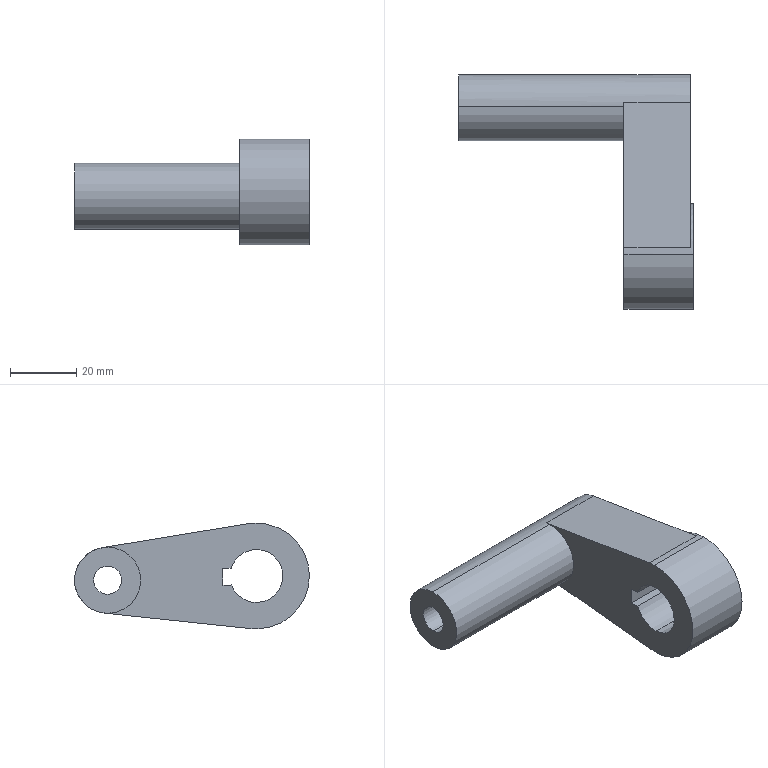Component | SolidWorks | 7Handle-1 | 1 solid | 21 faces | box 71 x 70.98 x 32 mm | volume 39259 mm3 | cylinder 11 | plane 10 | commonest cylinder face diameters 16 x3 12 x2 8.5 x2 32 x2 20 x2
STEP:
#1=CARTESIAN_POINT('',(-14.567,4.337,0.1854));
#2=VERTEX_POINT('',#1);
#3=CARTESIAN_POINT('',(-14.567,4.323,-0.2868));
#4=VERTEX_POINT('',#3);
#5=CARTESIAN_POINT('',(-14.567,4.33,-0.05068));
#6=DIRECTION('',(1.,0.,0.));
#7=DIRECTION('',(0.,0.02861,0.9996));
#8=AXIS2_PLACEMENT_3D('',#5,#6,#7);
#9=CIRCLE('',#8,0.2362);
#10=EDGE_CURVE('',#2,#4,#9,.T.);
#11=ORIENTED_EDGE('',*,*,#10,.F.);
#12=CARTESIAN_POINT('',(-12.047,4.337,0.1854));
#13=VERTEX_POINT('',#12);
#14=CARTESIAN_POINT('',(-15.471,4.337,0.1854));
#15=DIRECTION('',(1.,0.,0.));
#16=VECTOR('',#15,39.37);
#17=LINE('',#14,#16);
#18=EDGE_CURVE('',#2,#13,#17,.T.);
#19=ORIENTED_EDGE('',*,*,#18,.T.);
#20=CARTESIAN_POINT('',(-12.047,4.323,-0.2868));
#21=VERTEX_POINT('',#20);
#22=CARTESIAN_POINT('',(-12.047,4.33,-0.05068));
#23=DIRECTION('',(-1.,-0.,-0.));
#24=DIRECTION('',(0.,0.02861,0.9996));
#25=AXIS2_PLACEMENT_3D('',#22,#23,#24);
#26=CIRCLE('',#25,0.2362);
#27=EDGE_CURVE('',#21,#13,#26,.T.);
#28=ORIENTED_EDGE('',*,*,#27,.F.);
#29=CARTESIAN_POINT('',(-15.471,4.323,-0.2868));
#30=DIRECTION('',(1.,0.,0.));
#31=VECTOR('',#30,39.37);
#32=LINE('',#29,#31);
#33=EDGE_CURVE('',#4,#21,#32,.T.);
#34=ORIENTED_EDGE('',*,*,#33,.F.);
#35=EDGE_LOOP('',(#11,#19,#28,#34));
#36=FACE_OUTER_BOUND('',#35,.T.);
#37=CARTESIAN_POINT('',(-15.471,4.33,-0.05068));
#38=DIRECTION('',(1.,0.,0.));
#39=DIRECTION('',(0.,-0.02861,-0.9996));
#40=AXIS2_PLACEMENT_3D('',#37,#38,#39);
#41=CYLINDRICAL_SURFACE('',#40,0.2362);
#42=ADVANCED_FACE('',(#36),#41,.F.);
#43=CARTESIAN_POINT('',(-14.567,4.335,0.1166));
#44=VERTEX_POINT('',#43);
#45=CARTESIAN_POINT('',(-14.567,4.325,-0.2179));
#46=VERTEX_POINT('',#45);
#47=CARTESIAN_POINT('',(-14.567,4.33,-0.05068));
#48=DIRECTION('',(1.,0.,0.));
#49=DIRECTION('',(0.,0.02861,0.9996));
#50=AXIS2_PLACEMENT_3D('',#47,#48,#49);
#51=CIRCLE('',#50,0.1673);
#52=EDGE_CURVE('',#44,#46,#51,.T.);
#53=ORIENTED_EDGE('',*,*,#52,.T.);
#54=CARTESIAN_POINT('',(-14.803,4.325,-0.2179));
#55=VERTEX_POINT('',#54);
#56=CARTESIAN_POINT('',(-12.008,4.325,-0.2179));
#57=DIRECTION('',(-1.,-0.,-0.));
#58=VECTOR('',#57,39.37);
#59=LINE('',#56,#58);
#60=EDGE_CURVE('',#46,#55,#59,.T.);
#61=ORIENTED_EDGE('',*,*,#60,.T.);
#62=CARTESIAN_POINT('',(-14.803,4.335,0.1166));
#63=VERTEX_POINT('',#62);
#64=CARTESIAN_POINT('',(-14.803,4.33,-0.05068));
#65=DIRECTION('',(-1.,-0.,-0.));
#66=DIRECTION('',(0.,0.02861,0.9996));
#67=AXIS2_PLACEMENT_3D('',#64,#65,#66);
#68=CIRCLE('',#67,0.1673);
#69=EDGE_CURVE('',#55,#63,#68,.T.);
#70=ORIENTED_EDGE('',*,*,#69,.T.);
#71=CARTESIAN_POINT('',(-12.008,4.335,0.1166));
#72=DIRECTION('',(-1.,-0.,-0.));
#73=VECTOR('',#72,39.37);
#74=LINE('',#71,#73);
#75=EDGE_CURVE('',#44,#63,#74,.T.);
#76=ORIENTED_EDGE('',*,*,#75,.F.);
#77=EDGE_LOOP('',(#53,#61,#70,#76));
#78=FACE_OUTER_BOUND('',#77,.T.);
#79=CARTESIAN_POINT('',(-12.008,4.33,-0.05068));
#80=DIRECTION('',(-1.,-0.,-0.));
#81=DIRECTION('',(0.,0.02861,0.9996));
#82=AXIS2_PLACEMENT_3D('',#79,#80,#81);
#83=CYLINDRICAL_SURFACE('',#82,0.1673);
#84=ADVANCED_FACE('',(#78),#83,.F.);
#85=CARTESIAN_POINT('',(-12.008,2.55,-0.3148));
#86=VERTEX_POINT('',#85);
#87=CARTESIAN_POINT('',(-12.008,2.568,0.3148));
#88=VERTEX_POINT('',#87);
#89=CARTESIAN_POINT('',(-12.008,2.559,-0.));
#90=DIRECTION('',(-1.,-0.,-0.));
#91=DIRECTION('',(0.,0.02861,0.9996));
#92=AXIS2_PLACEMENT_3D('',#89,#90,#91);
#93=CIRCLE('',#92,0.315);
#94=EDGE_CURVE('',#86,#88,#93,.T.);
#95=ORIENTED_EDGE('',*,*,#94,.F.);
#96=CARTESIAN_POINT('',(-12.835,2.55,-0.3148));
#97=VERTEX_POINT('',#96);
#98=CARTESIAN_POINT('',(-12.008,2.55,-0.3148));
#99=DIRECTION('',(-1.,-0.,-0.));
#100=VECTOR('',#99,39.37);
#101=LINE('',#98,#100);
#102=EDGE_CURVE('',#86,#97,#101,.T.);
#103=ORIENTED_EDGE('',*,*,#102,.T.);
#104=CARTESIAN_POINT('',(-12.835,2.568,0.3148));
#105=VERTEX_POINT('',#104);
#106=CARTESIAN_POINT('',(-12.835,2.559,-0.));
#107=DIRECTION('',(-1.,-0.,-0.));
#108=DIRECTION('',(0.,0.02861,0.9996));
#109=AXIS2_PLACEMENT_3D('',#106,#107,#108);
#110=CIRCLE('',#109,0.315);
#111=EDGE_CURVE('',#97,#105,#110,.T.);
#112=ORIENTED_EDGE('',*,*,#111,.T.);
#113=CARTESIAN_POINT('',(-12.008,2.568,0.3148));
#114=DIRECTION('',(-1.,-0.,-0.));
#115=VECTOR('',#114,39.37);
#116=LINE('',#113,#115);
#117=EDGE_CURVE('',#88,#105,#116,.T.);
#118=ORIENTED_EDGE('',*,*,#117,.F.);
#119=EDGE_LOOP('',(#95,#103,#112,#118));
#120=FACE_OUTER_BOUND('',#119,.T.);
#121=CARTESIAN_POINT('',(-12.008,2.559,-0.));
#122=DIRECTION('',(-1.,-0.,-0.));
#123=DIRECTION('',(0.,0.02861,0.9996));
#124=AXIS2_PLACEMENT_3D('',#121,#122,#123);
#125=CYLINDRICAL_SURFACE('',#124,0.315);
#126=ADVANCED_FACE('',(#120),#125,.F.);
#127=CARTESIAN_POINT('',(-12.008,2.861,0.08983));
#128=VERTEX_POINT('',#127);
#129=CARTESIAN_POINT('',(-12.008,2.559,-0.));
#130=DIRECTION('',(-1.,-0.,-0.));
#131=DIRECTION('',(0.,0.02861,0.9996));
#132=AXIS2_PLACEMENT_3D('',#129,#130,#131);
#133=CIRCLE('',#132,0.315);
#134=EDGE_CURVE('',#88,#128,#133,.T.);
#135=ORIENTED_EDGE('',*,*,#134,.F.);
#136=ORIENTED_EDGE('',*,*,#117,.T.);
#137=CARTESIAN_POINT('',(-12.835,2.861,0.08983));
#138=VERTEX_POINT('',#137);
#139=CARTESIAN_POINT('',(-12.835,2.559,-0.));
#140=DIRECTION('',(-1.,-0.,-0.));
#141=DIRECTION('',(0.,0.02861,0.9996));
#142=AXIS2_PLACEMENT_3D('',#139,#140,#141);
#143=CIRCLE('',#142,0.315);
#144=EDGE_CURVE('',#105,#138,#143,.T.);
#145=ORIENTED_EDGE('',*,*,#144,.T.);
#146=CARTESIAN_POINT('',(-12.008,2.861,0.08983));
#147=DIRECTION('',(-1.,-0.,-0.));
#148=VECTOR('',#147,39.37);
#149=LINE('',#146,#148);
#150=EDGE_CURVE('',#128,#138,#149,.T.);
#151=ORIENTED_EDGE('',*,*,#150,.F.);
#152=EDGE_LOOP('',(#135,#136,#145,#151));
#153=FACE_OUTER_BOUND('',#152,.T.);
#154=CARTESIAN_POINT('',(-12.008,2.559,-0.));
#155=DIRECTION('',(-1.,-0.,-0.));
#156=DIRECTION('',(0.,0.02861,0.9996));
#157=AXIS2_PLACEMENT_3D('',#154,#155,#156);
#158=CYLINDRICAL_SURFACE('',#157,0.315);
#159=ADVANCED_FACE('',(#153),#158,.F.);
#160=CARTESIAN_POINT('',(-12.835,2.577,0.6297));
#161=VERTEX_POINT('',#160);
#162=CARTESIAN_POINT('',(-12.835,2.661,0.6216));
#163=VERTEX_POINT('',#162);
#164=CARTESIAN_POINT('',(-12.835,2.559,-0.));
#165=DIRECTION('',(-1.,-0.,-0.));
#166=DIRECTION('',(0.,0.02861,0.9996));
#167=AXIS2_PLACEMENT_3D('',#164,#165,#166);
#168=CIRCLE('',#167,0.6299);
#169=EDGE_CURVE('',#161,#163,#168,.T.);
#170=ORIENTED_EDGE('',*,*,#169,.F.);
#171=CARTESIAN_POINT('',(-12.008,2.577,0.6297));
#172=VERTEX_POINT('',#171);
#173=CARTESIAN_POINT('',(-12.835,2.577,0.6297));
#174=DIRECTION('',(1.,0.,0.));
#175=VECTOR('',#174,39.37);
#176=LINE('',#173,#175);
#177=EDGE_CURVE('',#161,#172,#176,.T.);
#178=ORIENTED_EDGE('',*,*,#177,.T.);
#179=CARTESIAN_POINT('',(-12.008,2.541,-0.6297));
#180=VERTEX_POINT('',#179);
#181=CARTESIAN_POINT('',(-12.008,2.559,-0.));
#182=DIRECTION('',(-1.,-0.,-0.));
#183=DIRECTION('',(0.,0.02861,0.9996));
#184=AXIS2_PLACEMENT_3D('',#181,#182,#183);
#185=CIRCLE('',#184,0.6299);
#186=EDGE_CURVE('',#172,#180,#185,.T.);
#187=ORIENTED_EDGE('',*,*,#186,.T.);
#188=CARTESIAN_POINT('',(-12.835,2.541,-0.6297));
#189=VERTEX_POINT('',#188);
#190=CARTESIAN_POINT('',(-12.835,2.541,-0.6297));
#191=DIRECTION('',(1.,0.,0.));
#192=VECTOR('',#191,39.37);
#193=LINE('',#190,#192);
#194=EDGE_CURVE('',#189,#180,#193,.T.);
#195=ORIENTED_EDGE('',*,*,#194,.F.);
#196=CARTESIAN_POINT('',(-12.835,2.625,-0.6264));
#197=VERTEX_POINT('',#196);
#198=CARTESIAN_POINT('',(-12.835,2.559,-0.));
#199=DIRECTION('',(-1.,-0.,-0.));
#200=DIRECTION('',(0.,0.02861,0.9996));
#201=AXIS2_PLACEMENT_3D('',#198,#199,#200);
#202=CIRCLE('',#201,0.6299);
#203=EDGE_CURVE('',#197,#189,#202,.T.);
#204=ORIENTED_EDGE('',*,*,#203,.F.);
#205=CARTESIAN_POINT('',(-12.047,2.625,-0.6264));
#206=VERTEX_POINT('',#205);
#207=CARTESIAN_POINT('',(-12.835,2.625,-0.6264));
#208=DIRECTION('',(1.,0.,0.));
#209=VECTOR('',#208,39.37);
#210=LINE('',#207,#209);
#211=EDGE_CURVE('',#197,#206,#210,.T.);
#212=ORIENTED_EDGE('',*,*,#211,.T.);
#213=CARTESIAN_POINT('',(-12.047,2.661,0.6216));
#214=VERTEX_POINT('',#213);
#215=CARTESIAN_POINT('',(-12.047,2.559,-0.));
#216=DIRECTION('',(-1.,-0.,-0.));
#217=DIRECTION('',(0.,0.02861,0.9996));
#218=AXIS2_PLACEMENT_3D('',#215,#216,#217);
#219=CIRCLE('',#218,0.6299);
#220=EDGE_CURVE('',#214,#206,#219,.T.);
#221=ORIENTED_EDGE('',*,*,#220,.F.);
#222=CARTESIAN_POINT('',(-12.835,2.661,0.6216));
#223=DIRECTION('',(1.,0.,0.));
#224=VECTOR('',#223,39.37);
#225=LINE('',#222,#224);
#226=EDGE_CURVE('',#163,#214,#225,.T.);
#227=ORIENTED_EDGE('',*,*,#226,.F.);
#228=EDGE_LOOP('',(#170,#178,#187,#195,#204,#212,#221,#227));
#229=FACE_OUTER_BOUND('',#228,.T.);
#230=CARTESIAN_POINT('',(-12.835,2.559,-0.));
#231=DIRECTION('',(1.,0.,0.));
#232=DIRECTION('',(0.,-0.02861,-0.9996));
#233=AXIS2_PLACEMENT_3D('',#230,#231,#232);
#234=CYLINDRICAL_SURFACE('',#233,0.6299);
#235=ADVANCED_FACE('',(#229),#234,.T.);
#236=CARTESIAN_POINT('',(-14.803,4.341,0.3429));
#237=VERTEX_POINT('',#236);
#238=CARTESIAN_POINT('',(-14.803,4.319,-0.4442));
#239=VERTEX_POINT('',#238);
#240=CARTESIAN_POINT('',(-14.803,4.33,-0.05068));
#241=DIRECTION('',(-1.,-0.,-0.));
#242=DIRECTION('',(0.,0.02861,0.9996));
#243=AXIS2_PLACEMENT_3D('',#240,#241,#242);
#244=CIRCLE('',#243,0.3937);
#245=EDGE_CURVE('',#237,#239,#244,.T.);
#246=ORIENTED_EDGE('',*,*,#245,.F.);
#247=CARTESIAN_POINT('',(-12.835,4.341,0.3429));
#248=VERTEX_POINT('',#247);
#249=CARTESIAN_POINT('',(-14.803,4.341,0.3429));
#250=DIRECTION('',(1.,0.,0.));
#251=VECTOR('',#250,39.37);
#252=LINE('',#249,#251);
#253=EDGE_CURVE('',#237,#248,#252,.T.);
#254=ORIENTED_EDGE('',*,*,#253,.T.);
#255=CARTESIAN_POINT('',(-12.835,4.394,0.3378));
#256=VERTEX_POINT('',#255);
#257=CARTESIAN_POINT('',(-12.835,4.33,-0.05068));
#258=DIRECTION('',(-1.,-0.,-0.));
#259=DIRECTION('',(0.,0.02861,0.9996));
#260=AXIS2_PLACEMENT_3D('',#257,#258,#259);
#261=CIRCLE('',#260,0.3937);
#262=EDGE_CURVE('',#248,#256,#261,.T.);
#263=ORIENTED_EDGE('',*,*,#262,.T.);
#264=CARTESIAN_POINT('',(-12.047,4.394,0.3378));
#265=VERTEX_POINT('',#264);
#266=CARTESIAN_POINT('',(-12.835,4.394,0.3378));
#267=DIRECTION('',(1.,0.,0.));
#268=VECTOR('',#267,39.37);
#269=LINE('',#266,#268);
#270=EDGE_CURVE('',#256,#265,#269,.T.);
#271=ORIENTED_EDGE('',*,*,#270,.T.);
#272=CARTESIAN_POINT('',(-12.047,4.371,-0.4422));
#273=VERTEX_POINT('',#272);
#274=CARTESIAN_POINT('',(-12.047,4.33,-0.05068));
#275=DIRECTION('',(-1.,-0.,-0.));
#276=DIRECTION('',(0.,0.02861,0.9996));
#277=AXIS2_PLACEMENT_3D('',#274,#275,#276);
#278=CIRCLE('',#277,0.3937);
#279=EDGE_CURVE('',#265,#273,#278,.T.);
#280=ORIENTED_EDGE('',*,*,#279,.T.);
#281=CARTESIAN_POINT('',(-12.835,4.371,-0.4422));
#282=VERTEX_POINT('',#281);
#283=CARTESIAN_POINT('',(-12.835,4.371,-0.4422));
#284=DIRECTION('',(1.,0.,0.));
#285=VECTOR('',#284,39.37);
#286=LINE('',#283,#285);
#287=EDGE_CURVE('',#282,#273,#286,.T.);
#288=ORIENTED_EDGE('',*,*,#287,.F.);
#289=CARTESIAN_POINT('',(-12.835,4.319,-0.4442));
#290=VERTEX_POINT('',#289);
#291=CARTESIAN_POINT('',(-12.835,4.33,-0.05068));
#292=DIRECTION('',(-1.,-0.,-0.));
#293=DIRECTION('',(0.,0.02861,0.9996));
#294=AXIS2_PLACEMENT_3D('',#291,#292,#293);
#295=CIRCLE('',#294,0.3937);
#296=EDGE_CURVE('',#282,#290,#295,.T.);
#297=ORIENTED_EDGE('',*,*,#296,.T.);
#298=CARTESIAN_POINT('',(-14.803,4.319,-0.4442));
#299=DIRECTION('',(1.,0.,0.));
#300=VECTOR('',#299,39.37);
#301=LINE('',#298,#300);
#302=EDGE_CURVE('',#239,#290,#301,.T.);
#303=ORIENTED_EDGE('',*,*,#302,.F.);
#304=EDGE_LOOP('',(#246,#254,#263,#271,#280,#288,#297,#303));
#305=FACE_OUTER_BOUND('',#304,.T.);
#306=CARTESIAN_POINT('',(-14.803,4.33,-0.05068));
#307=DIRECTION('',(1.,0.,0.));
#308=DIRECTION('',(0.,-0.02861,-0.9996));
#309=AXIS2_PLACEMENT_3D('',#306,#307,#308);
#310=CYLINDRICAL_SURFACE('',#309,0.3937);
#311=ADVANCED_FACE('',(#305),#310,.T.);
#312=CARTESIAN_POINT('',(-12.835,4.371,-0.4422));
#313=DIRECTION('',(0.,-0.9945,-0.1049));
#314=VECTOR('',#313,39.37);
#315=LINE('',#312,#314);
#316=EDGE_CURVE('',#282,#197,#315,.T.);
#317=ORIENTED_EDGE('',*,*,#316,.T.);
#318=ORIENTED_EDGE('',*,*,#203,.T.);
#319=CARTESIAN_POINT('',(-12.835,2.559,-0.));
#320=DIRECTION('',(-1.,-0.,-0.));
#321=DIRECTION('',(0.,0.02861,0.9996));
#322=AXIS2_PLACEMENT_3D('',#319,#320,#321);
#323=CIRCLE('',#322,0.6299);
#324=EDGE_CURVE('',#189,#161,#323,.T.);
#325=ORIENTED_EDGE('',*,*,#324,.T.);
#326=ORIENTED_EDGE('',*,*,#169,.T.);
#327=CARTESIAN_POINT('',(-12.835,4.394,0.3378));
#328=DIRECTION('',(0.,-0.9869,0.1616));
#329=VECTOR('',#328,39.37);
#330=LINE('',#327,#329);
#331=EDGE_CURVE('',#256,#163,#330,.T.);
#332=ORIENTED_EDGE('',*,*,#331,.F.);
#333=ORIENTED_EDGE('',*,*,#262,.F.);
#334=CARTESIAN_POINT('',(-12.835,4.33,-0.05068));
#335=DIRECTION('',(-1.,-0.,-0.));
#336=DIRECTION('',(0.,0.02861,0.9996));
#337=AXIS2_PLACEMENT_3D('',#334,#335,#336);
#338=CIRCLE('',#337,0.3937);
#339=EDGE_CURVE('',#290,#248,#338,.T.);
#340=ORIENTED_EDGE('',*,*,#339,.F.);
#341=ORIENTED_EDGE('',*,*,#296,.F.);
#342=EDGE_LOOP('',(#317,#318,#325,#326,#332,#333,#340,#341));
#343=FACE_OUTER_BOUND('',#342,.T.);
#344=CARTESIAN_POINT('',(-12.835,2.958,-0.1099));
#345=VERTEX_POINT('',#344);
#346=CARTESIAN_POINT('',(-12.835,2.855,-0.1069));
#347=VERTEX_POINT('',#346);
#348=CARTESIAN_POINT('',(-12.835,4.327,-0.1491));
#349=DIRECTION('',(0.,-0.9996,0.02861));
#350=VECTOR('',#349,39.37);
#351=LINE('',#348,#350);
#352=EDGE_CURVE('',#345,#347,#351,.T.);
#353=ORIENTED_EDGE('',*,*,#352,.F.);
#354=CARTESIAN_POINT('',(-12.835,2.963,0.0869));
#355=VERTEX_POINT('',#354);
#356=CARTESIAN_POINT('',(-12.835,2.96,-0.01149));
#357=DIRECTION('',(-0.,0.02861,0.9996));
#358=VECTOR('',#357,39.37);
#359=LINE('',#356,#358);
#360=EDGE_CURVE('',#345,#355,#359,.T.);
#361=ORIENTED_EDGE('',*,*,#360,.T.);
#362=CARTESIAN_POINT('',(-12.835,4.333,0.0477));
#363=DIRECTION('',(0.,-0.9996,0.02861));
#364=VECTOR('',#363,39.37);
#365=LINE('',#362,#364);
#366=EDGE_CURVE('',#355,#138,#365,.T.);
#367=ORIENTED_EDGE('',*,*,#366,.T.);
#368=ORIENTED_EDGE('',*,*,#144,.F.);
#369=ORIENTED_EDGE('',*,*,#111,.F.);
#370=CARTESIAN_POINT('',(-12.835,2.559,-0.));
#371=DIRECTION('',(-1.,-0.,-0.));
#372=DIRECTION('',(0.,0.02861,0.9996));
#373=AXIS2_PLACEMENT_3D('',#370,#371,#372);
#374=CIRCLE('',#373,0.315);
#375=EDGE_CURVE('',#347,#97,#374,.T.);
#376=ORIENTED_EDGE('',*,*,#375,.F.);
#377=EDGE_LOOP('',(#353,#361,#367,#368,#369,#376));
#378=FACE_BOUND('',#377,.T.);
#379=CARTESIAN_POINT('',(-12.835,4.33,-0.05068));
#380=DIRECTION('',(-1.,-0.,-0.));
#381=DIRECTION('',(-0.,0.02861,0.9996));
#382=AXIS2_PLACEMENT_3D('',#379,#380,#381);
#383=PLANE('',#382);
#384=ADVANCED_FACE('',(#343,#378),#383,.T.);
#385=CARTESIAN_POINT('',(-12.008,2.559,-0.));
#386=DIRECTION('',(-1.,-0.,-0.));
#387=DIRECTION('',(0.,0.02861,0.9996));
#388=AXIS2_PLACEMENT_3D('',#385,#386,#387);
#389=CIRCLE('',#388,0.6299);
#390=EDGE_CURVE('',#180,#172,#389,.T.);
#391=ORIENTED_EDGE('',*,*,#390,.F.);
#392=ORIENTED_EDGE('',*,*,#186,.F.);
#393=EDGE_LOOP('',(#391,#392));
#394=FACE_OUTER_BOUND('',#393,.T.);
#395=CARTESIAN_POINT('',(-12.008,2.958,-0.1099));
#396=VERTEX_POINT('',#395);
#397=CARTESIAN_POINT('',(-12.008,2.963,0.0869));
#398=VERTEX_POINT('',#397);
#399=CARTESIAN_POINT('',(-12.008,2.96,-0.01149));
#400=DIRECTION('',(-0.,0.02861,0.9996));
#401=VECTOR('',#400,39.37);
#402=LINE('',#399,#401);
#403=EDGE_CURVE('',#396,#398,#402,.T.);
#404=ORIENTED_EDGE('',*,*,#403,.F.);
#405=CARTESIAN_POINT('',(-12.008,2.855,-0.1069));
#406=VERTEX_POINT('',#405);
#407=CARTESIAN_POINT('',(-12.008,4.327,-0.1491));
#408=DIRECTION('',(0.,-0.9996,0.02861));
#409=VECTOR('',#408,39.37);
#410=LINE('',#407,#409);
#411=EDGE_CURVE('',#396,#406,#410,.T.);
#412=ORIENTED_EDGE('',*,*,#411,.T.);
#413=CARTESIAN_POINT('',(-12.008,2.559,-0.));
#414=DIRECTION('',(-1.,-0.,-0.));
#415=DIRECTION('',(0.,0.02861,0.9996));
#416=AXIS2_PLACEMENT_3D('',#413,#414,#415);
#417=CIRCLE('',#416,0.315);
#418=EDGE_CURVE('',#406,#86,#417,.T.);
#419=ORIENTED_EDGE('',*,*,#418,.T.);
#420=ORIENTED_EDGE('',*,*,#94,.T.);
#421=ORIENTED_EDGE('',*,*,#134,.T.);
#422=CARTESIAN_POINT('',(-12.008,4.333,0.0477));
#423=DIRECTION('',(0.,-0.9996,0.02861));
#424=VECTOR('',#423,39.37);
#425=LINE('',#422,#424);
#426=EDGE_CURVE('',#398,#128,#425,.T.);
#427=ORIENTED_EDGE('',*,*,#426,.F.);
#428=EDGE_LOOP('',(#404,#412,#419,#420,#421,#427));
#429=FACE_BOUND('',#428,.T.);
#430=CARTESIAN_POINT('',(-12.008,4.33,-0.05068));
#431=DIRECTION('',(-1.,-0.,-0.));
#432=DIRECTION('',(-0.,0.02861,0.9996));
#433=AXIS2_PLACEMENT_3D('',#430,#431,#432);
#434=PLANE('',#433);
#435=ADVANCED_FACE('',(#394,#429),#434,.F.);
#436=ORIENTED_EDGE('',*,*,#253,.F.);
#437=CARTESIAN_POINT('',(-14.803,4.33,-0.05068));
#438=DIRECTION('',(-1.,-0.,-0.));
#439=DIRECTION('',(0.,0.02861,0.9996));
#440=AXIS2_PLACEMENT_3D('',#437,#438,#439);
#441=CIRCLE('',#440,0.3937);
#442=EDGE_CURVE('',#239,#237,#441,.T.);
#443=ORIENTED_EDGE('',*,*,#442,.F.);
#444=ORIENTED_EDGE('',*,*,#302,.T.);
#445=ORIENTED_EDGE('',*,*,#339,.T.);
#446=EDGE_LOOP('',(#436,#443,#444,#445));
#447=FACE_OUTER_BOUND('',#446,.T.);
#448=CARTESIAN_POINT('',(-14.803,4.33,-0.05068));
#449=DIRECTION('',(1.,0.,0.));
#450=DIRECTION('',(0.,-0.02861,-0.9996));
#451=AXIS2_PLACEMENT_3D('',#448,#449,#450);
#452=CYLINDRICAL_SURFACE('',#451,0.3937);
#453=ADVANCED_FACE('',(#447),#452,.T.);
#454=CARTESIAN_POINT('',(-14.803,4.33,-0.05068));
#455=DIRECTION('',(-1.,-0.,-0.));
#456=DIRECTION('',(0.,0.02861,0.9996));
#457=AXIS2_PLACEMENT_3D('',#454,#455,#456);
#458=CIRCLE('',#457,0.1673);
#459=EDGE_CURVE('',#63,#55,#458,.T.);
#460=ORIENTED_EDGE('',*,*,#459,.F.);
#461=ORIENTED_EDGE('',*,*,#69,.F.);
#462=EDGE_LOOP('',(#460,#461));
#463=FACE_BOUND('',#462,.T.);
#464=ORIENTED_EDGE('',*,*,#442,.T.);
#465=ORIENTED_EDGE('',*,*,#245,.T.);
#466=EDGE_LOOP('',(#464,#465));
#467=FACE_OUTER_BOUND('',#466,.T.);
#468=CARTESIAN_POINT('',(-14.803,4.33,-0.05068));
#469=DIRECTION('',(-1.,-0.,-0.));
#470=DIRECTION('',(-0.,0.02861,0.9996));
#471=AXIS2_PLACEMENT_3D('',#468,#469,#470);
#472=PLANE('',#471);
#473=ADVANCED_FACE('',(#463,#467),#472,.T.);
#474=ORIENTED_EDGE('',*,*,#27,.T.);
#475=CARTESIAN_POINT('',(-12.047,4.33,-0.05068));
#476=DIRECTION('',(-1.,-0.,-0.));
#477=DIRECTION('',(0.,0.02861,0.9996));
#478=AXIS2_PLACEMENT_3D('',#475,#476,#477);
#479=CIRCLE('',#478,0.2362);
#480=EDGE_CURVE('',#13,#21,#479,.T.);
#481=ORIENTED_EDGE('',*,*,#480,.T.);
#482=EDGE_LOOP('',(#474,#481));
#483=FACE_BOUND('',#482,.T.);
#484=CARTESIAN_POINT('',(-12.047,4.394,0.3378));
#485=DIRECTION('',(0.,-0.9869,0.1616));
#486=VECTOR('',#485,39.37);
#487=LINE('',#484,#486);
#488=EDGE_CURVE('',#265,#214,#487,.T.);
#489=ORIENTED_EDGE('',*,*,#488,.T.);
#490=ORIENTED_EDGE('',*,*,#220,.T.);
#491=CARTESIAN_POINT('',(-12.047,4.371,-0.4422));
#492=DIRECTION('',(0.,-0.9945,-0.1049));
#493=VECTOR('',#492,39.37);
#494=LINE('',#491,#493);
#495=EDGE_CURVE('',#273,#206,#494,.T.);
#496=ORIENTED_EDGE('',*,*,#495,.F.);
#497=ORIENTED_EDGE('',*,*,#279,.F.);
#498=EDGE_LOOP('',(#489,#490,#496,#497));
#499=FACE_OUTER_BOUND('',#498,.T.);
#500=CARTESIAN_POINT('',(-12.047,4.33,-0.05068));
#501=DIRECTION('',(-1.,-0.,-0.));
#502=DIRECTION('',(-0.,0.02861,0.9996));
#503=AXIS2_PLACEMENT_3D('',#500,#501,#502);
#504=PLANE('',#503);
#505=ADVANCED_FACE('',(#483,#499),#504,.F.);
#506=ORIENTED_EDGE('',*,*,#495,.T.);
#507=ORIENTED_EDGE('',*,*,#211,.F.);
#508=ORIENTED_EDGE('',*,*,#316,.F.);
#509=ORIENTED_EDGE('',*,*,#287,.T.);
#510=EDGE_LOOP('',(#506,#507,#508,#509));
#511=FACE_OUTER_BOUND('',#510,.T.);
#512=CARTESIAN_POINT('',(-12.835,4.371,-0.4422));
#513=DIRECTION('',(-0.,-0.1049,0.9945));
#514=DIRECTION('',(-0.,0.9945,0.1049));
#515=AXIS2_PLACEMENT_3D('',#512,#513,#514);
#516=PLANE('',#515);
#517=ADVANCED_FACE('',(#511),#516,.F.);
#518=ORIENTED_EDGE('',*,*,#177,.F.);
#519=ORIENTED_EDGE('',*,*,#324,.F.);
#520=ORIENTED_EDGE('',*,*,#194,.T.);
#521=ORIENTED_EDGE('',*,*,#390,.T.);
#522=EDGE_LOOP('',(#518,#519,#520,#521));
#523=FACE_OUTER_BOUND('',#522,.T.);
#524=CARTESIAN_POINT('',(-12.835,2.559,-0.));
#525=DIRECTION('',(1.,0.,0.));
#526=DIRECTION('',(0.,-0.02861,-0.9996));
#527=AXIS2_PLACEMENT_3D('',#524,#525,#526);
#528=CYLINDRICAL_SURFACE('',#527,0.6299);
#529=ADVANCED_FACE('',(#523),#528,.T.);
#530=ORIENTED_EDGE('',*,*,#488,.F.);
#531=ORIENTED_EDGE('',*,*,#270,.F.);
#532=ORIENTED_EDGE('',*,*,#331,.T.);
#533=ORIENTED_EDGE('',*,*,#226,.T.);
#534=EDGE_LOOP('',(#530,#531,#532,#533));
#535=FACE_OUTER_BOUND('',#534,.T.);
#536=CARTESIAN_POINT('',(-12.835,4.394,0.3378));
#537=DIRECTION('',(-0.,0.1616,0.9869));
#538=DIRECTION('',(-0.,0.9869,-0.1616));
#539=AXIS2_PLACEMENT_3D('',#536,#537,#538);
#540=PLANE('',#539);
#541=ADVANCED_FACE('',(#535),#540,.T.);
#542=ORIENTED_EDGE('',*,*,#102,.F.);
#543=ORIENTED_EDGE('',*,*,#418,.F.);
#544=CARTESIAN_POINT('',(-12.008,2.855,-0.1069));
#545=DIRECTION('',(-1.,-0.,-0.));
#546=VECTOR('',#545,39.37);
#547=LINE('',#544,#546);
#548=EDGE_CURVE('',#406,#347,#547,.T.);
#549=ORIENTED_EDGE('',*,*,#548,.T.);
#550=ORIENTED_EDGE('',*,*,#375,.T.);
#551=EDGE_LOOP('',(#542,#543,#549,#550));
#552=FACE_OUTER_BOUND('',#551,.T.);
#553=CARTESIAN_POINT('',(-12.008,2.559,-0.));
#554=DIRECTION('',(-1.,-0.,-0.));
#555=DIRECTION('',(0.,0.02861,0.9996));
#556=AXIS2_PLACEMENT_3D('',#553,#554,#555);
#557=CYLINDRICAL_SURFACE('',#556,0.315);
#558=ADVANCED_FACE('',(#552),#557,.F.);
#559=ORIENTED_EDGE('',*,*,#352,.T.);
#560=ORIENTED_EDGE('',*,*,#548,.F.);
#561=ORIENTED_EDGE('',*,*,#411,.F.);
#562=CARTESIAN_POINT('',(-12.008,2.958,-0.1099));
#563=DIRECTION('',(-1.,-0.,-0.));
#564=VECTOR('',#563,39.37);
#565=LINE('',#562,#564);
#566=EDGE_CURVE('',#396,#345,#565,.T.);
#567=ORIENTED_EDGE('',*,*,#566,.T.);
#568=EDGE_LOOP('',(#559,#560,#561,#567));
#569=FACE_OUTER_BOUND('',#568,.T.);
#570=CARTESIAN_POINT('',(-12.008,4.327,-0.1491));
#571=DIRECTION('',(0.,-0.02861,-0.9996));
#572=DIRECTION('',(-1.,-0.,-0.));
#573=AXIS2_PLACEMENT_3D('',#570,#571,#572);
#574=PLANE('',#573);
#575=ADVANCED_FACE('',(#569),#574,.F.);
#576=CARTESIAN_POINT('',(-12.008,2.963,0.0869));
#577=DIRECTION('',(-1.,-0.,-0.));
#578=VECTOR('',#577,39.37);
#579=LINE('',#576,#578);
#580=EDGE_CURVE('',#398,#355,#579,.T.);
#581=ORIENTED_EDGE('',*,*,#580,.F.);
#582=ORIENTED_EDGE('',*,*,#426,.T.);
#583=ORIENTED_EDGE('',*,*,#150,.T.);
#584=ORIENTED_EDGE('',*,*,#366,.F.);
#585=EDGE_LOOP('',(#581,#582,#583,#584));
#586=FACE_OUTER_BOUND('',#585,.T.);
#587=CARTESIAN_POINT('',(-12.008,4.333,0.0477));
#588=DIRECTION('',(0.,-0.02861,-0.9996));
#589=DIRECTION('',(-1.,-0.,-0.));
#590=AXIS2_PLACEMENT_3D('',#587,#588,#589);
#591=PLANE('',#590);
#592=ADVANCED_FACE('',(#586),#591,.T.);
#593=ORIENTED_EDGE('',*,*,#566,.F.);
#594=ORIENTED_EDGE('',*,*,#403,.T.);
#595=ORIENTED_EDGE('',*,*,#580,.T.);
#596=ORIENTED_EDGE('',*,*,#360,.F.);
#597=EDGE_LOOP('',(#593,#594,#595,#596));
#598=FACE_OUTER_BOUND('',#597,.T.);
#599=CARTESIAN_POINT('',(-12.008,2.96,-0.01149));
#600=DIRECTION('',(0.,-0.9996,0.02861));
#601=DIRECTION('',(1.,0.,0.));
#602=AXIS2_PLACEMENT_3D('',#599,#600,#601);
#603=PLANE('',#602);
#604=ADVANCED_FACE('',(#598),#603,.T.);
#605=ORIENTED_EDGE('',*,*,#60,.F.);
#606=CARTESIAN_POINT('',(-14.567,4.33,-0.05068));
#607=DIRECTION('',(1.,0.,0.));
#608=DIRECTION('',(0.,0.02861,0.9996));
#609=AXIS2_PLACEMENT_3D('',#606,#607,#608);
#610=CIRCLE('',#609,0.1673);
#611=EDGE_CURVE('',#46,#44,#610,.T.);
#612=ORIENTED_EDGE('',*,*,#611,.T.);
#613=ORIENTED_EDGE('',*,*,#75,.T.);
#614=ORIENTED_EDGE('',*,*,#459,.T.);
#615=EDGE_LOOP('',(#605,#612,#613,#614));
#616=FACE_OUTER_BOUND('',#615,.T.);
#617=CARTESIAN_POINT('',(-12.008,4.33,-0.05068));
#618=DIRECTION('',(-1.,-0.,-0.));
#619=DIRECTION('',(0.,0.02861,0.9996));
#620=AXIS2_PLACEMENT_3D('',#617,#618,#619);
#621=CYLINDRICAL_SURFACE('',#620,0.1673);
#622=ADVANCED_FACE('',(#616),#621,.F.);
#623=ORIENTED_EDGE('',*,*,#18,.F.);
#624=CARTESIAN_POINT('',(-14.567,4.33,-0.05068));
#625=DIRECTION('',(1.,0.,0.));
#626=DIRECTION('',(0.,0.02861,0.9996));
#627=AXIS2_PLACEMENT_3D('',#624,#625,#626);
#628=CIRCLE('',#627,0.2362);
#629=EDGE_CURVE('',#4,#2,#628,.T.);
#630=ORIENTED_EDGE('',*,*,#629,.F.);
#631=ORIENTED_EDGE('',*,*,#33,.T.);
#632=ORIENTED_EDGE('',*,*,#480,.F.);
#633=EDGE_LOOP('',(#623,#630,#631,#632));
#634=FACE_OUTER_BOUND('',#633,.T.);
#635=CARTESIAN_POINT('',(-15.471,4.33,-0.05068));
#636=DIRECTION('',(1.,0.,0.));
#637=DIRECTION('',(0.,-0.02861,-0.9996));
#638=AXIS2_PLACEMENT_3D('',#635,#636,#637);
#639=CYLINDRICAL_SURFACE('',#638,0.2362);
#640=ADVANCED_FACE('',(#634),#639,.F.);
#641=ORIENTED_EDGE('',*,*,#629,.T.);
#642=ORIENTED_EDGE('',*,*,#10,.T.);
#643=EDGE_LOOP('',(#641,#642));
#644=FACE_OUTER_BOUND('',#643,.T.);
#645=ORIENTED_EDGE('',*,*,#52,.F.);
#646=ORIENTED_EDGE('',*,*,#611,.F.);
#647=EDGE_LOOP('',(#645,#646));
#648=FACE_BOUND('',#647,.T.);
#649=CARTESIAN_POINT('',(-14.567,4.33,-0.05068));
#650=DIRECTION('',(-1.,-0.,-0.));
#651=DIRECTION('',(-0.,0.02861,0.9996));
#652=AXIS2_PLACEMENT_3D('',#649,#650,#651);
#653=PLANE('',#652);
#654=ADVANCED_FACE('',(#644,#648),#653,.F.);
#655=CLOSED_SHELL('',(#42,#84,#126,#159,#235,#311,#384,#435,#453,#473,#505,#517,#529,#541,#558,#575,#592,#604,#622,#640,#654));
#656=MANIFOLD_SOLID_BREP('',#655);
#657=CARTESIAN_POINT('',(0.,0.,0.));
#658=DIRECTION('',(0.,0.,1.));
#659=DIRECTION('',(1.,0.,0.));
#660=AXIS2_PLACEMENT_3D('',#657,#658,#659);
#661=(LENGTH_UNIT()NAMED_UNIT(*)SI_UNIT($,.METRE.));
#662=LENGTH_MEASURE_WITH_UNIT(LENGTH_MEASURE(0.0254),#661);
#663=DIMENSIONAL_EXPONENTS(1.,0.,0.,0.,0.,0.,0.);
#664=(CONVERSION_BASED_UNIT('',#662)LENGTH_UNIT()NAMED_UNIT(#663));
#665=UNCERTAINTY_MEASURE_WITH_UNIT(LENGTH_MEASURE(0.00001),#664,'','');
#666=(NAMED_UNIT(*)PLANE_ANGLE_UNIT()SI_UNIT($,.RADIAN.));
#667=(NAMED_UNIT(*)SI_UNIT($,.STERADIAN.)SOLID_ANGLE_UNIT());
#668=(GEOMETRIC_REPRESENTATION_CONTEXT(3)GLOBAL_UNCERTAINTY_ASSIGNED_CONTEXT((#665))GLOBAL_UNIT_ASSIGNED_CONTEXT((#664,#666,#667))REPRESENTATION_CONTEXT('',''));
#669=ADVANCED_BREP_SHAPE_REPRESENTATION('',(#656,#660),#668);
#670=COLOUR_RGB('',0.7922,0.8196,0.9333);
#671=FILL_AREA_STYLE_COLOUR('',#670);
#672=FILL_AREA_STYLE('',(#671));
#673=SURFACE_STYLE_FILL_AREA(#672);
#674=SURFACE_SIDE_STYLE('',(#673));
#675=SURFACE_STYLE_USAGE(.BOTH.,#674);
#676=PRESENTATION_STYLE_ASSIGNMENT((#675));
#677=STYLED_ITEM('',(#676),#656);
#678=(LENGTH_UNIT()NAMED_UNIT(*)SI_UNIT($,.METRE.));
#679=LENGTH_MEASURE_WITH_UNIT(LENGTH_MEASURE(0.0254),#678);
#680=DIMENSIONAL_EXPONENTS(1.,0.,0.,0.,0.,0.,0.);
#681=(CONVERSION_BASED_UNIT('',#679)LENGTH_UNIT()NAMED_UNIT(#680));
#682=UNCERTAINTY_MEASURE_WITH_UNIT(LENGTH_MEASURE(0.00001),#681,'','');
#683=(NAMED_UNIT(*)PLANE_ANGLE_UNIT()SI_UNIT($,.RADIAN.));
#684=(NAMED_UNIT(*)SI_UNIT($,.STERADIAN.)SOLID_ANGLE_UNIT());
#685=(GEOMETRIC_REPRESENTATION_CONTEXT(3)GLOBAL_UNCERTAINTY_ASSIGNED_CONTEXT((#682))GLOBAL_UNIT_ASSIGNED_CONTEXT((#681,#683,#684))REPRESENTATION_CONTEXT('',''));
#686=MECHANICAL_DESIGN_GEOMETRIC_PRESENTATION_REPRESENTATION('',(#677),#685);
#687=PRESENTATION_LAYER_ASSIGNMENT('','',(#677));